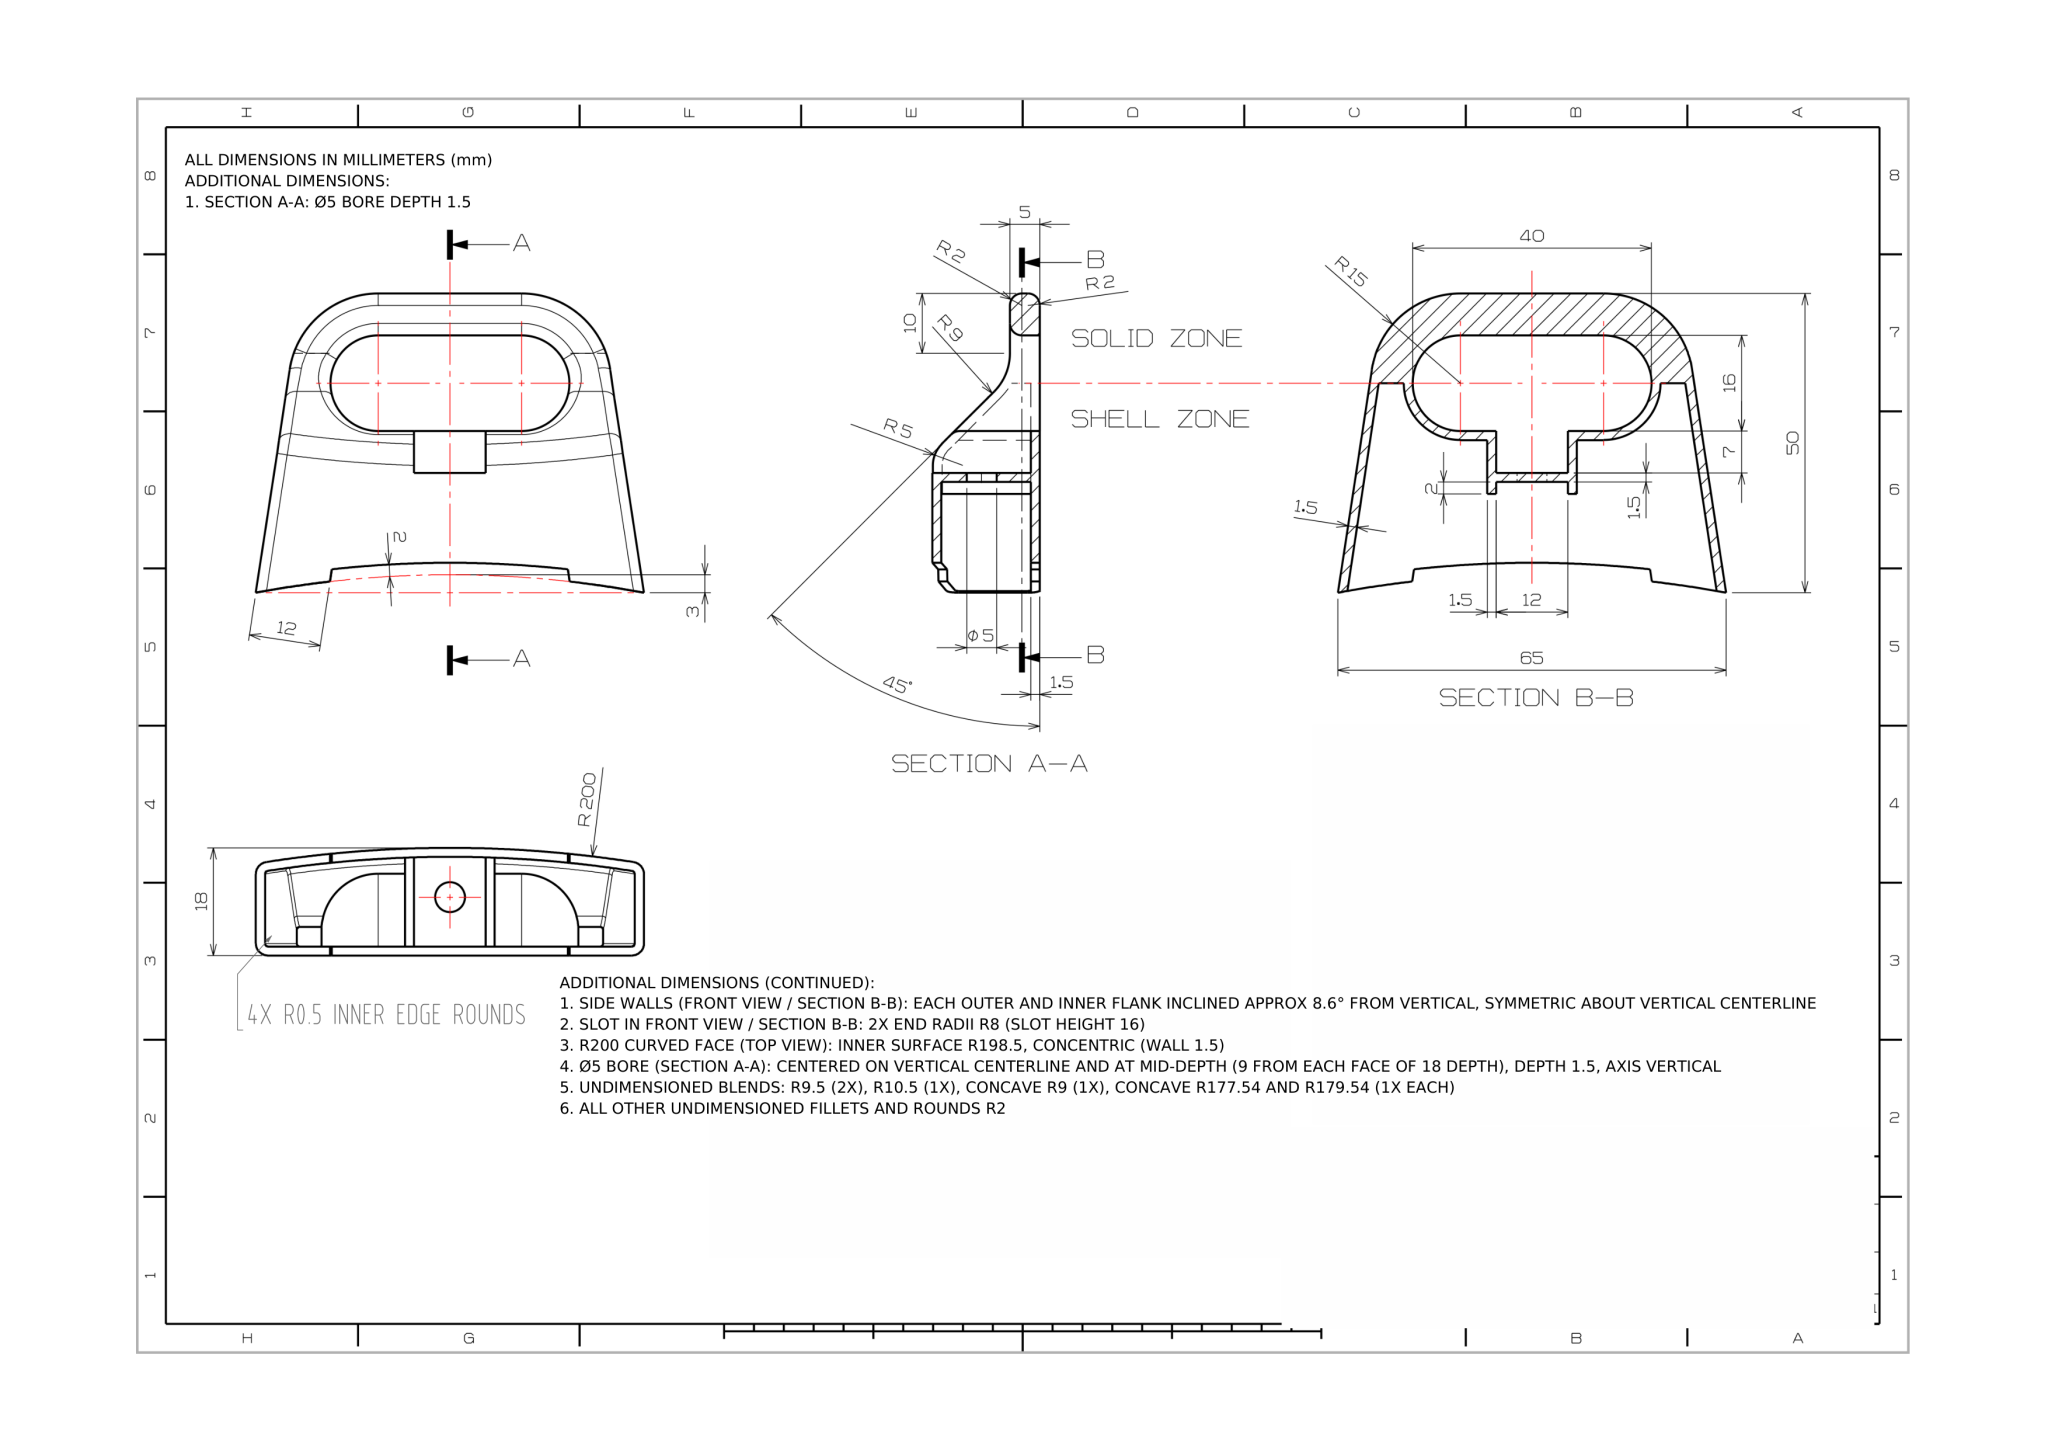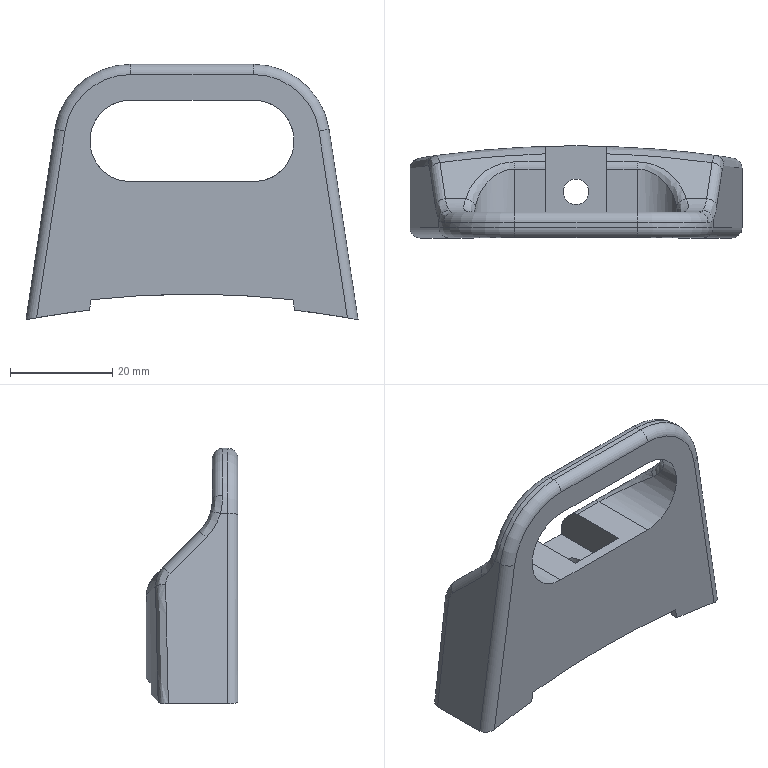Part | NX | mm | 1 solid | 91 faces | box 65 x 18 x 50 mm | volume 9082 mm3 | plane 33 | cylinder 30 | spline 22 | torus 6 | commonest cylinder face diameters 4 x9 1 x4 355.083 x2 359.083 x2 16 x2 18 x2 19 x2 21 x2